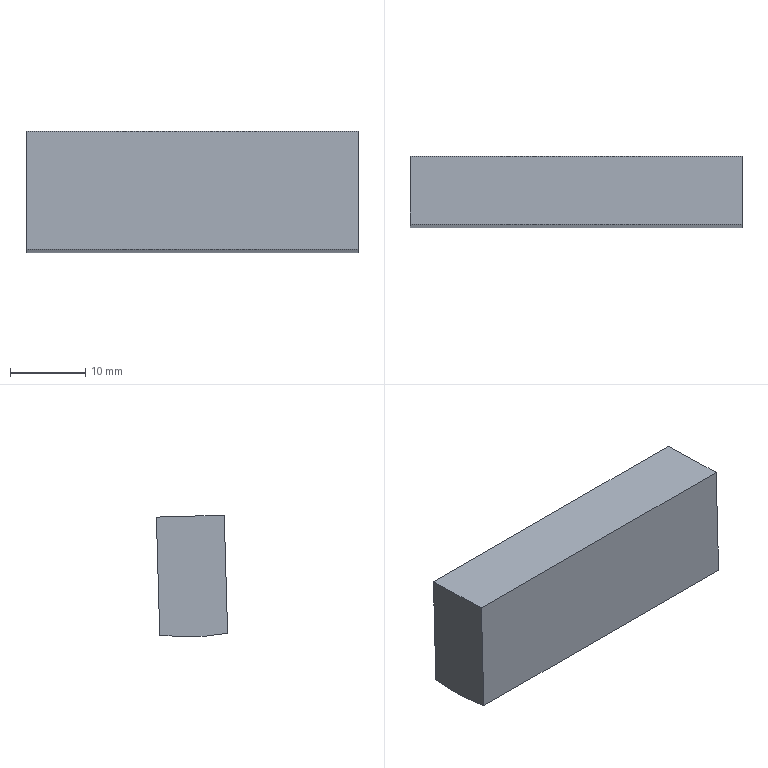Component | NX | VANE_2 | 1 solid | 6 faces | box 44 x 9.44 x 16.13 mm | volume 6290 mm3 | plane 5 | cylinder 1 | commonest cylinder face diameters 58 x1
STEP:
#1=CARTESIAN_POINT('',(0.,0.,0.));
#2=DIRECTION('',(0.,0.,1.));
#3=DIRECTION('',(1.,0.,0.));
#4=AXIS2_PLACEMENT_3D('',#1,#2,#3);
#5=CARTESIAN_POINT('',(-2.,-4.855,-2.832));
#6=VERTEX_POINT('',#5);
#7=CARTESIAN_POINT('',(-2.,-5.302,-18.475));
#8=VERTEX_POINT('',#7);
#9=CARTESIAN_POINT('',(-2.,-4.855,-2.832));
#10=DIRECTION('',(0.,-0.0286,-0.9996));
#11=VECTOR('',#10,1.);
#12=LINE('',#9,#11);
#13=CARTESIAN_POINT('',(42.,-4.855,-2.832));
#14=DIRECTION('',(0.,0.9996,-0.0286));
#15=DIRECTION('',(0.,0.0286,0.9996));
#16=AXIS2_PLACEMENT_3D('',#13,#14,#15);
#17=PLANE('',#16);
#18=CARTESIAN_POINT('',(0.,-44.));
#19=DIRECTION('',(-1.,0.));
#20=VECTOR('',#19,1.);
#21=LINE('',#18,#20);
#22=(GEOMETRIC_REPRESENTATION_CONTEXT(2)PARAMETRIC_REPRESENTATION_CONTEXT()REPRESENTATION_CONTEXT('',''));
#23=DEFINITIONAL_REPRESENTATION('',(#21),#22);
#24=PCURVE('',#17,#23);
#25=CARTESIAN_POINT('',(-2.,0.01527,10.034));
#26=DIRECTION('',(1.,0.,0.));
#27=DIRECTION('',(0.,0.0286,0.9996));
#28=AXIS2_PLACEMENT_3D('',#25,#26,#27);
#29=PLANE('',#28);
#30=CARTESIAN_POINT('',(-13.,4.5));
#31=DIRECTION('',(-1.,0.));
#32=VECTOR('',#31,1.);
#33=LINE('',#30,#32);
#34=(GEOMETRIC_REPRESENTATION_CONTEXT(2)PARAMETRIC_REPRESENTATION_CONTEXT()REPRESENTATION_CONTEXT('',''));
#35=DEFINITIONAL_REPRESENTATION('',(#33),#34);
#36=PCURVE('',#29,#35);
#37=SURFACE_CURVE('',#12,(#24,#36),.PCURVE_S1.);
#38=EDGE_CURVE('',#6,#8,#37,.T.);
#39=ORIENTED_EDGE('',*,*,#38,.T.);
#40=CARTESIAN_POINT('',(42.,-5.302,-18.475));
#41=VERTEX_POINT('',#40);
#42=CARTESIAN_POINT('',(42.,-5.302,-18.475));
#43=DIRECTION('',(-1.,0.,0.));
#44=VECTOR('',#43,1.);
#45=LINE('',#42,#44);
#46=CARTESIAN_POINT('',(-15.649,0.));
#47=DIRECTION('',(0.,-1.));
#48=VECTOR('',#47,1.);
#49=LINE('',#46,#48);
#50=(GEOMETRIC_REPRESENTATION_CONTEXT(2)PARAMETRIC_REPRESENTATION_CONTEXT()REPRESENTATION_CONTEXT('',''));
#51=DEFINITIONAL_REPRESENTATION('',(#49),#50);
#52=PCURVE('',#17,#51);
#53=CARTESIAN_POINT('',(42.,0.01527,10.034));
#54=DIRECTION('',(-1.,0.,0.));
#55=DIRECTION('',(0.,-0.0286,-0.9996));
#56=AXIS2_PLACEMENT_3D('',#53,#54,#55);
#57=CYLINDRICAL_SURFACE('',#56,29.);
#58=CARTESIAN_POINT('',(6.439,0.));
#59=DIRECTION('',(0.,1.));
#60=VECTOR('',#59,1.);
#61=LINE('',#58,#60);
#62=(GEOMETRIC_REPRESENTATION_CONTEXT(2)PARAMETRIC_REPRESENTATION_CONTEXT()REPRESENTATION_CONTEXT('',''));
#63=DEFINITIONAL_REPRESENTATION('',(#61),#62);
#64=PCURVE('',#57,#63);
#65=SURFACE_CURVE('',#45,(#52,#64),.PCURVE_S1.);
#66=EDGE_CURVE('',#41,#8,#65,.T.);
#67=ORIENTED_EDGE('',*,*,#66,.F.);
#68=CARTESIAN_POINT('',(42.,-4.855,-2.832));
#69=VERTEX_POINT('',#68);
#70=CARTESIAN_POINT('',(42.,-4.855,-2.832));
#71=DIRECTION('',(0.,-0.0286,-0.9996));
#72=VECTOR('',#71,1.);
#73=LINE('',#70,#72);
#74=CARTESIAN_POINT('',(0.,0.));
#75=DIRECTION('',(-1.,0.));
#76=VECTOR('',#75,1.);
#77=LINE('',#74,#76);
#78=(GEOMETRIC_REPRESENTATION_CONTEXT(2)PARAMETRIC_REPRESENTATION_CONTEXT()REPRESENTATION_CONTEXT('',''));
#79=DEFINITIONAL_REPRESENTATION('',(#77),#78);
#80=PCURVE('',#17,#79);
#81=CARTESIAN_POINT('',(42.,0.01527,10.034));
#82=DIRECTION('',(1.,0.,0.));
#83=DIRECTION('',(0.,0.0286,0.9996));
#84=AXIS2_PLACEMENT_3D('',#81,#82,#83);
#85=PLANE('',#84);
#86=CARTESIAN_POINT('',(-13.,4.5));
#87=DIRECTION('',(-1.,0.));
#88=VECTOR('',#87,1.);
#89=LINE('',#86,#88);
#90=(GEOMETRIC_REPRESENTATION_CONTEXT(2)PARAMETRIC_REPRESENTATION_CONTEXT()REPRESENTATION_CONTEXT('',''));
#91=DEFINITIONAL_REPRESENTATION('',(#89),#90);
#92=PCURVE('',#85,#91);
#93=SURFACE_CURVE('',#73,(#80,#92),.PCURVE_S1.);
#94=EDGE_CURVE('',#69,#41,#93,.T.);
#95=ORIENTED_EDGE('',*,*,#94,.F.);
#96=CARTESIAN_POINT('',(42.,-4.855,-2.832));
#97=DIRECTION('',(-1.,0.,0.));
#98=VECTOR('',#97,1.);
#99=LINE('',#96,#98);
#100=CARTESIAN_POINT('',(0.,0.));
#101=DIRECTION('',(0.,-1.));
#102=VECTOR('',#101,1.);
#103=LINE('',#100,#102);
#104=(GEOMETRIC_REPRESENTATION_CONTEXT(2)PARAMETRIC_REPRESENTATION_CONTEXT()REPRESENTATION_CONTEXT('',''));
#105=DEFINITIONAL_REPRESENTATION('',(#103),#104);
#106=PCURVE('',#17,#105);
#107=CARTESIAN_POINT('',(42.,-0.3566,-2.961));
#108=DIRECTION('',(0.,-0.0286,-0.9996));
#109=DIRECTION('',(1.,0.,0.));
#110=AXIS2_PLACEMENT_3D('',#107,#108,#109);
#111=PLANE('',#110);
#112=CARTESIAN_POINT('',(0.,4.5));
#113=DIRECTION('',(-1.,0.));
#114=VECTOR('',#113,1.);
#115=LINE('',#112,#114);
#116=(GEOMETRIC_REPRESENTATION_CONTEXT(2)PARAMETRIC_REPRESENTATION_CONTEXT()REPRESENTATION_CONTEXT('',''));
#117=DEFINITIONAL_REPRESENTATION('',(#115),#116);
#118=PCURVE('',#111,#117);
#119=SURFACE_CURVE('',#99,(#106,#118),.PCURVE_S1.);
#120=EDGE_CURVE('',#69,#6,#119,.T.);
#121=ORIENTED_EDGE('',*,*,#120,.T.);
#122=EDGE_LOOP('',(#39,#67,#95,#121));
#123=FACE_BOUND('',#122,.T.);
#124=ADVANCED_FACE('',(#123),#17,.F.);
#125=CARTESIAN_POINT('',(-2.,3.694,-18.732));
#126=VERTEX_POINT('',#125);
#127=CARTESIAN_POINT('',(-2.,0.01527,10.034));
#128=DIRECTION('',(1.,0.,0.));
#129=DIRECTION('',(0.,-0.9996,0.0286));
#130=AXIS2_PLACEMENT_3D('',#127,#128,#129);
#131=CIRCLE('',#130,29.);
#132=CARTESIAN_POINT('',(7.854,44.));
#133=DIRECTION('',(-1.,0.));
#134=VECTOR('',#133,1.);
#135=LINE('',#132,#134);
#136=(GEOMETRIC_REPRESENTATION_CONTEXT(2)PARAMETRIC_REPRESENTATION_CONTEXT()REPRESENTATION_CONTEXT('',''));
#137=DEFINITIONAL_REPRESENTATION('',(#135),#136);
#138=PCURVE('',#57,#137);
#139=CARTESIAN_POINT('',(0.,0.));
#140=DIRECTION('',(0.,1.));
#141=AXIS2_PLACEMENT_2D('',#139,#140);
#142=CIRCLE('',#141,29.);
#143=(GEOMETRIC_REPRESENTATION_CONTEXT(2)PARAMETRIC_REPRESENTATION_CONTEXT()REPRESENTATION_CONTEXT('',''));
#144=DEFINITIONAL_REPRESENTATION('',(#142),#143);
#145=PCURVE('',#29,#144);
#146=SURFACE_CURVE('',#131,(#138,#145),.PCURVE_S1.);
#147=EDGE_CURVE('',#8,#126,#146,.T.);
#148=ORIENTED_EDGE('',*,*,#147,.T.);
#149=CARTESIAN_POINT('',(42.,3.694,-18.732));
#150=VERTEX_POINT('',#149);
#151=CARTESIAN_POINT('',(42.,3.694,-18.732));
#152=DIRECTION('',(-1.,0.,0.));
#153=VECTOR('',#152,1.);
#154=LINE('',#151,#153);
#155=CARTESIAN_POINT('',(6.127,0.));
#156=DIRECTION('',(0.,1.));
#157=VECTOR('',#156,1.);
#158=LINE('',#155,#157);
#159=(GEOMETRIC_REPRESENTATION_CONTEXT(2)PARAMETRIC_REPRESENTATION_CONTEXT()REPRESENTATION_CONTEXT('',''));
#160=DEFINITIONAL_REPRESENTATION('',(#158),#159);
#161=PCURVE('',#57,#160);
#162=CARTESIAN_POINT('',(42.,3.694,-18.732));
#163=DIRECTION('',(0.,-0.9996,0.0286));
#164=DIRECTION('',(0.,-0.0286,-0.9996));
#165=AXIS2_PLACEMENT_3D('',#162,#163,#164);
#166=PLANE('',#165);
#167=CARTESIAN_POINT('',(-0.,0.));
#168=DIRECTION('',(0.,-1.));
#169=VECTOR('',#168,1.);
#170=LINE('',#167,#169);
#171=(GEOMETRIC_REPRESENTATION_CONTEXT(2)PARAMETRIC_REPRESENTATION_CONTEXT()REPRESENTATION_CONTEXT('',''));
#172=DEFINITIONAL_REPRESENTATION('',(#170),#171);
#173=PCURVE('',#166,#172);
#174=SURFACE_CURVE('',#154,(#161,#173),.PCURVE_S1.);
#175=EDGE_CURVE('',#150,#126,#174,.T.);
#176=ORIENTED_EDGE('',*,*,#175,.F.);
#177=CARTESIAN_POINT('',(42.,0.01527,10.034));
#178=DIRECTION('',(1.,0.,0.));
#179=DIRECTION('',(0.,-0.9996,0.0286));
#180=AXIS2_PLACEMENT_3D('',#177,#178,#179);
#181=CIRCLE('',#180,29.);
#182=CARTESIAN_POINT('',(7.854,0.));
#183=DIRECTION('',(-1.,0.));
#184=VECTOR('',#183,1.);
#185=LINE('',#182,#184);
#186=(GEOMETRIC_REPRESENTATION_CONTEXT(2)PARAMETRIC_REPRESENTATION_CONTEXT()REPRESENTATION_CONTEXT('',''));
#187=DEFINITIONAL_REPRESENTATION('',(#185),#186);
#188=PCURVE('',#57,#187);
#189=CARTESIAN_POINT('',(0.,0.));
#190=DIRECTION('',(0.,1.));
#191=AXIS2_PLACEMENT_2D('',#189,#190);
#192=CIRCLE('',#191,29.);
#193=(GEOMETRIC_REPRESENTATION_CONTEXT(2)PARAMETRIC_REPRESENTATION_CONTEXT()REPRESENTATION_CONTEXT('',''));
#194=DEFINITIONAL_REPRESENTATION('',(#192),#193);
#195=PCURVE('',#85,#194);
#196=SURFACE_CURVE('',#181,(#188,#195),.PCURVE_S1.);
#197=EDGE_CURVE('',#41,#150,#196,.T.);
#198=ORIENTED_EDGE('',*,*,#197,.F.);
#199=ORIENTED_EDGE('',*,*,#66,.T.);
#200=EDGE_LOOP('',(#148,#176,#198,#199));
#201=FACE_BOUND('',#200,.T.);
#202=ADVANCED_FACE('',(#201),#57,.T.);
#203=CARTESIAN_POINT('',(-2.,4.142,-3.09));
#204=VERTEX_POINT('',#203);
#205=CARTESIAN_POINT('',(-2.,3.694,-18.732));
#206=DIRECTION('',(0.,0.0286,0.9996));
#207=VECTOR('',#206,1.);
#208=LINE('',#205,#207);
#209=CARTESIAN_POINT('',(0.,-44.));
#210=DIRECTION('',(-1.,0.));
#211=VECTOR('',#210,1.);
#212=LINE('',#209,#211);
#213=(GEOMETRIC_REPRESENTATION_CONTEXT(2)PARAMETRIC_REPRESENTATION_CONTEXT()REPRESENTATION_CONTEXT('',''));
#214=DEFINITIONAL_REPRESENTATION('',(#212),#213);
#215=PCURVE('',#166,#214);
#216=CARTESIAN_POINT('',(-28.649,-4.5));
#217=DIRECTION('',(1.,0.));
#218=VECTOR('',#217,1.);
#219=LINE('',#216,#218);
#220=(GEOMETRIC_REPRESENTATION_CONTEXT(2)PARAMETRIC_REPRESENTATION_CONTEXT()REPRESENTATION_CONTEXT('',''));
#221=DEFINITIONAL_REPRESENTATION('',(#219),#220);
#222=PCURVE('',#29,#221);
#223=SURFACE_CURVE('',#208,(#215,#222),.PCURVE_S1.);
#224=EDGE_CURVE('',#126,#204,#223,.T.);
#225=ORIENTED_EDGE('',*,*,#224,.T.);
#226=CARTESIAN_POINT('',(42.,4.142,-3.09));
#227=VERTEX_POINT('',#226);
#228=CARTESIAN_POINT('',(42.,4.142,-3.09));
#229=DIRECTION('',(-1.,0.,0.));
#230=VECTOR('',#229,1.);
#231=LINE('',#228,#230);
#232=CARTESIAN_POINT('',(-15.649,0.));
#233=DIRECTION('',(0.,-1.));
#234=VECTOR('',#233,1.);
#235=LINE('',#232,#234);
#236=(GEOMETRIC_REPRESENTATION_CONTEXT(2)PARAMETRIC_REPRESENTATION_CONTEXT()REPRESENTATION_CONTEXT('',''));
#237=DEFINITIONAL_REPRESENTATION('',(#235),#236);
#238=PCURVE('',#166,#237);
#239=CARTESIAN_POINT('',(0.,-4.5));
#240=DIRECTION('',(-1.,0.));
#241=VECTOR('',#240,1.);
#242=LINE('',#239,#241);
#243=(GEOMETRIC_REPRESENTATION_CONTEXT(2)PARAMETRIC_REPRESENTATION_CONTEXT()REPRESENTATION_CONTEXT('',''));
#244=DEFINITIONAL_REPRESENTATION('',(#242),#243);
#245=PCURVE('',#111,#244);
#246=SURFACE_CURVE('',#231,(#238,#245),.PCURVE_S1.);
#247=EDGE_CURVE('',#227,#204,#246,.T.);
#248=ORIENTED_EDGE('',*,*,#247,.F.);
#249=CARTESIAN_POINT('',(42.,3.694,-18.732));
#250=DIRECTION('',(0.,0.0286,0.9996));
#251=VECTOR('',#250,1.);
#252=LINE('',#249,#251);
#253=CARTESIAN_POINT('',(0.,0.));
#254=DIRECTION('',(-1.,0.));
#255=VECTOR('',#254,1.);
#256=LINE('',#253,#255);
#257=(GEOMETRIC_REPRESENTATION_CONTEXT(2)PARAMETRIC_REPRESENTATION_CONTEXT()REPRESENTATION_CONTEXT('',''));
#258=DEFINITIONAL_REPRESENTATION('',(#256),#257);
#259=PCURVE('',#166,#258);
#260=CARTESIAN_POINT('',(-28.649,-4.5));
#261=DIRECTION('',(1.,0.));
#262=VECTOR('',#261,1.);
#263=LINE('',#260,#262);
#264=(GEOMETRIC_REPRESENTATION_CONTEXT(2)PARAMETRIC_REPRESENTATION_CONTEXT()REPRESENTATION_CONTEXT('',''));
#265=DEFINITIONAL_REPRESENTATION('',(#263),#264);
#266=PCURVE('',#85,#265);
#267=SURFACE_CURVE('',#252,(#259,#266),.PCURVE_S1.);
#268=EDGE_CURVE('',#150,#227,#267,.T.);
#269=ORIENTED_EDGE('',*,*,#268,.F.);
#270=ORIENTED_EDGE('',*,*,#175,.T.);
#271=EDGE_LOOP('',(#225,#248,#269,#270));
#272=FACE_BOUND('',#271,.T.);
#273=ADVANCED_FACE('',(#272),#166,.F.);
#274=CARTESIAN_POINT('',(-2.,-0.3566,-2.961));
#275=DIRECTION('',(0.,-0.9996,0.0286));
#276=VECTOR('',#275,1.);
#277=LINE('',#274,#276);
#278=CARTESIAN_POINT('',(-44.,0.));
#279=DIRECTION('',(0.,1.));
#280=VECTOR('',#279,1.);
#281=LINE('',#278,#280);
#282=(GEOMETRIC_REPRESENTATION_CONTEXT(2)PARAMETRIC_REPRESENTATION_CONTEXT()REPRESENTATION_CONTEXT('',''));
#283=DEFINITIONAL_REPRESENTATION('',(#281),#282);
#284=PCURVE('',#111,#283);
#285=CARTESIAN_POINT('',(-13.,-0.));
#286=DIRECTION('',(0.,1.));
#287=VECTOR('',#286,1.);
#288=LINE('',#285,#287);
#289=(GEOMETRIC_REPRESENTATION_CONTEXT(2)PARAMETRIC_REPRESENTATION_CONTEXT()REPRESENTATION_CONTEXT('',''));
#290=DEFINITIONAL_REPRESENTATION('',(#288),#289);
#291=PCURVE('',#29,#290);
#292=SURFACE_CURVE('',#277,(#284,#291),.PCURVE_S1.);
#293=EDGE_CURVE('',#204,#6,#292,.T.);
#294=ORIENTED_EDGE('',*,*,#293,.T.);
#295=ORIENTED_EDGE('',*,*,#120,.F.);
#296=CARTESIAN_POINT('',(42.,4.142,-3.09));
#297=DIRECTION('',(0.,-0.9996,0.0286));
#298=VECTOR('',#297,1.);
#299=LINE('',#296,#298);
#300=CARTESIAN_POINT('',(0.,-4.5));
#301=DIRECTION('',(0.,1.));
#302=VECTOR('',#301,1.);
#303=LINE('',#300,#302);
#304=(GEOMETRIC_REPRESENTATION_CONTEXT(2)PARAMETRIC_REPRESENTATION_CONTEXT()REPRESENTATION_CONTEXT('',''));
#305=DEFINITIONAL_REPRESENTATION('',(#303),#304);
#306=PCURVE('',#111,#305);
#307=CARTESIAN_POINT('',(-13.,-4.5));
#308=DIRECTION('',(0.,1.));
#309=VECTOR('',#308,1.);
#310=LINE('',#307,#309);
#311=(GEOMETRIC_REPRESENTATION_CONTEXT(2)PARAMETRIC_REPRESENTATION_CONTEXT()REPRESENTATION_CONTEXT('',''));
#312=DEFINITIONAL_REPRESENTATION('',(#310),#311);
#313=PCURVE('',#85,#312);
#314=SURFACE_CURVE('',#299,(#306,#313),.PCURVE_S1.);
#315=EDGE_CURVE('',#227,#69,#314,.T.);
#316=ORIENTED_EDGE('',*,*,#315,.F.);
#317=ORIENTED_EDGE('',*,*,#247,.T.);
#318=EDGE_LOOP('',(#294,#295,#316,#317));
#319=FACE_BOUND('',#318,.T.);
#320=ADVANCED_FACE('',(#319),#111,.F.);
#321=ORIENTED_EDGE('',*,*,#94,.T.);
#322=ORIENTED_EDGE('',*,*,#197,.T.);
#323=ORIENTED_EDGE('',*,*,#268,.T.);
#324=ORIENTED_EDGE('',*,*,#315,.T.);
#325=EDGE_LOOP('',(#321,#322,#323,#324));
#326=FACE_BOUND('',#325,.T.);
#327=ADVANCED_FACE('',(#326),#85,.T.);
#328=ORIENTED_EDGE('',*,*,#38,.F.);
#329=ORIENTED_EDGE('',*,*,#293,.F.);
#330=ORIENTED_EDGE('',*,*,#224,.F.);
#331=ORIENTED_EDGE('',*,*,#147,.F.);
#332=EDGE_LOOP('',(#328,#329,#330,#331));
#333=FACE_BOUND('',#332,.T.);
#334=ADVANCED_FACE('',(#333),#29,.F.);
#335=CLOSED_SHELL('',(#124,#202,#273,#320,#327,#334));
#336=MANIFOLD_SOLID_BREP('',#335);
#337=(LENGTH_UNIT()NAMED_UNIT(*)SI_UNIT(.MILLI.,.METRE.));
#338=UNCERTAINTY_MEASURE_WITH_UNIT(LENGTH_MEASURE(0.0000001),#337,'','');
#339=(NAMED_UNIT(*)PLANE_ANGLE_UNIT()SI_UNIT($,.RADIAN.));
#340=(NAMED_UNIT(*)SI_UNIT($,.STERADIAN.)SOLID_ANGLE_UNIT());
#341=(GEOMETRIC_REPRESENTATION_CONTEXT(3)GLOBAL_UNCERTAINTY_ASSIGNED_CONTEXT((#338))GLOBAL_UNIT_ASSIGNED_CONTEXT((#337,#339,#340))REPRESENTATION_CONTEXT('',''));
#342=ADVANCED_BREP_SHAPE_REPRESENTATION('',(#4,#336),#341);